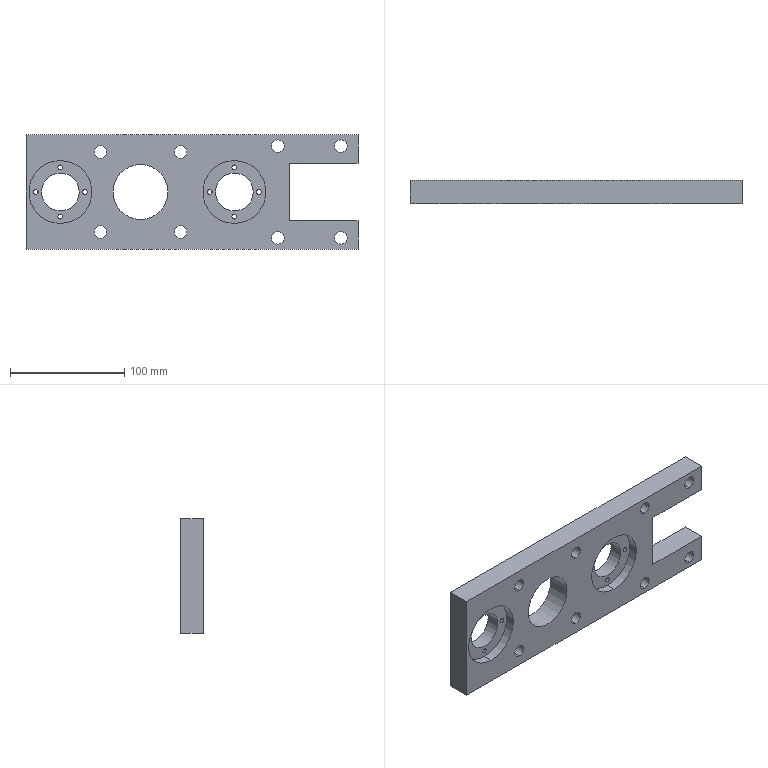Component | SolidWorks | SHYTJ-01-07-01CylinderMountingPlate-1 | 1 solid | 66 faces | box 290 x 20 x 100 mm | volume 401718 mm3 | cylinder 50 | plane 16 | commonest cylinder face diameters 4.2 x16 11 x16 18 x8 55 x4 33 x4 48 x2
build123d program:
from build123d import *

# Parameters (mm, degrees)
SKETCH1_W                                         = 290
SKETCH1_H                                         = 20
BOSS_EXTRUDE1_DEPTH                               = 100
HOLE_SIZE_ACCORDING_TO_TYPE_OF_SOCKET_D           = 11
HOLE_SIZE_ACCORDING_TO_TYPE_OF_SOCKET_CBORE_D     = 18
HOLE_SIZE_ACCORDING_TO_TYPE_OF_SOCKET_CBORE_DEPTH = 11
SKETCH4_R                                         = 24
CUT_EXTRUDE1_DEPTH                                = 308.409
F_11_0_11_DIAMETER_HOLE1_D                        = 11
SKETCH7_R                                         = 16.5
CUT_EXTRUDE2_DEPTH                                = 308.409
SKETCH8_R                                         = 27.5
CUT_EXTRUDE3_DEPTH                                = 8
M5_TAPPED_HOLE1_D                                 = 4.2
LPATTERN1_COUNT                                   = 2
LPATTERN1_PITCH                                   = 152
SKETCH15_W                                        = 60
SKETCH15_H                                        = 50
CUT_EXTRUDE4_DEPTH                                = 308.409


with BuildPart() as part:
    # Sketch1 → Boss-Extrude1 (new body)
    with BuildSketch(Plane.XY):
        with Locations((145, 10)):
            Rectangle(SKETCH1_W, SKETCH1_H)
    extrude(amount=BOSS_EXTRUDE1_DEPTH)

    # Hole Size _according to_ type of socket (through all)
    with Locations(Plane(origin=(0, 20, 0), x_dir=(1, 0, 0), z_dir=(0, 1, 0))):
        with Locations((220, -10), (220, -90), (275, -10), (275, -90)):
            CounterBoreHole(HOLE_SIZE_ACCORDING_TO_TYPE_OF_SOCKET_D / 2, HOLE_SIZE_ACCORDING_TO_TYPE_OF_SOCKET_CBORE_D / 2, HOLE_SIZE_ACCORDING_TO_TYPE_OF_SOCKET_CBORE_DEPTH)

    # Sketch4 → Cut-Extrude1 (cut, through all)
    with BuildSketch(Plane(origin=(0, 20, 0), x_dir=(1, 0, 0), z_dir=(0, 1, 0))):
        with Locations(Location((100, -50, 0), (0, 0, 180))):
            Circle(SKETCH4_R)
    extrude(amount=-CUT_EXTRUDE1_DEPTH, mode=Mode.SUBTRACT)

    # 11.0 _11_ Diameter Hole1 (through all)
    with Locations(Plane.XZ):
        with Locations((65, 15), (65, 85), (135, 85), (135, 15)):
            Hole(F_11_0_11_DIAMETER_HOLE1_D / 2)

    # Sketch7 → Cut-Extrude2 (cut, through all)
    with BuildSketch(Plane(origin=(0, 20, 0), x_dir=(1, 0, 0), z_dir=(0, 1, 0))):
        with Locations(Location((30, -50, 0), (0, 0, 180))):
            Circle(SKETCH7_R)
        with Locations(Location((182, -50, 0), (0, 0, 180))):
            Circle(SKETCH7_R)
    extrude(amount=-CUT_EXTRUDE2_DEPTH, mode=Mode.SUBTRACT)

    # Sketch8 → Cut-Extrude3 (cut)
    with BuildSketch(Plane.XZ):
        with Locations(Location((30, 50, 0), (0, 0, 270))):
            Circle(SKETCH8_R)
        with Locations(Location((182, 50, 0), (0, 0, 270))):
            Circle(SKETCH8_R)
    extrude(amount=-CUT_EXTRUDE3_DEPTH, mode=Mode.SUBTRACT)

    # M5 Tapped Hole1 (through all)
    with Locations(Plane(origin=(0, 8, 0), x_dir=(-1, 0, 0), z_dir=(0, -1, 0))):
        with Locations((-30, -71.5), (-30, -28.5), (-51.5, -50), (-8.5, -50)):
            m5_tapped_hole1 = Hole(M5_TAPPED_HOLE1_D / 2)

    # LPattern1: M5 Tapped Hole1 ×2
    with Locations(*[(i * LPATTERN1_PITCH, 0, 0) for i in range(1, LPATTERN1_COUNT)]):
        add(m5_tapped_hole1, mode=Mode.SUBTRACT)

    # Sketch15 → Cut-Extrude4 (cut, through all)
    with BuildSketch(Plane(origin=(0, 20, 0), x_dir=(1, 0, 0), z_dir=(0, 1, 0))):
        with Locations((260, -50)):
            Rectangle(SKETCH15_W, SKETCH15_H)
    extrude(amount=-CUT_EXTRUDE4_DEPTH, mode=Mode.SUBTRACT)


solid = part.part

# Placed as in the assembly
solid = solid.moved(Location((-80.116, -20.361, 220), (0, 0, 0)))